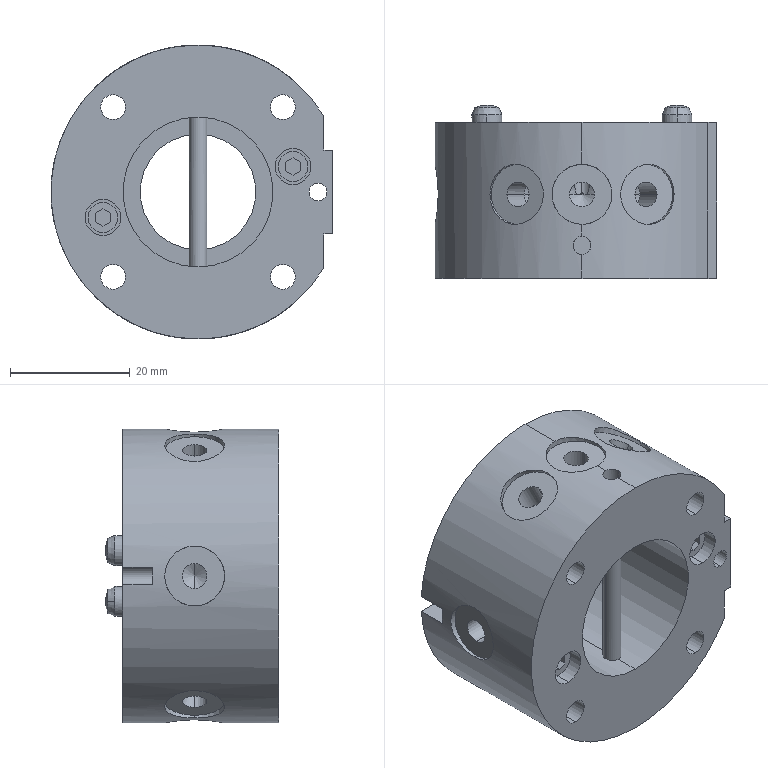Component | SolidWorks | F-SWS-005-000-000-1_F-SCHUNK-0302308 SWA-005-000-000, 00-1_F-_SCHUNK-SWA 005-000-000-parts, 01-1 | 1 solid | 206 faces | box 47 x 29.01 x 49 mm | volume 33247 mm3 | cylinder 100 | cone 64 | plane 40 | spline 2 | commonest cylinder face diameters 4.134 x22 6 x16 10 x14 2.6 x12 3 x11 2.459 x8 5 x8 49 x3